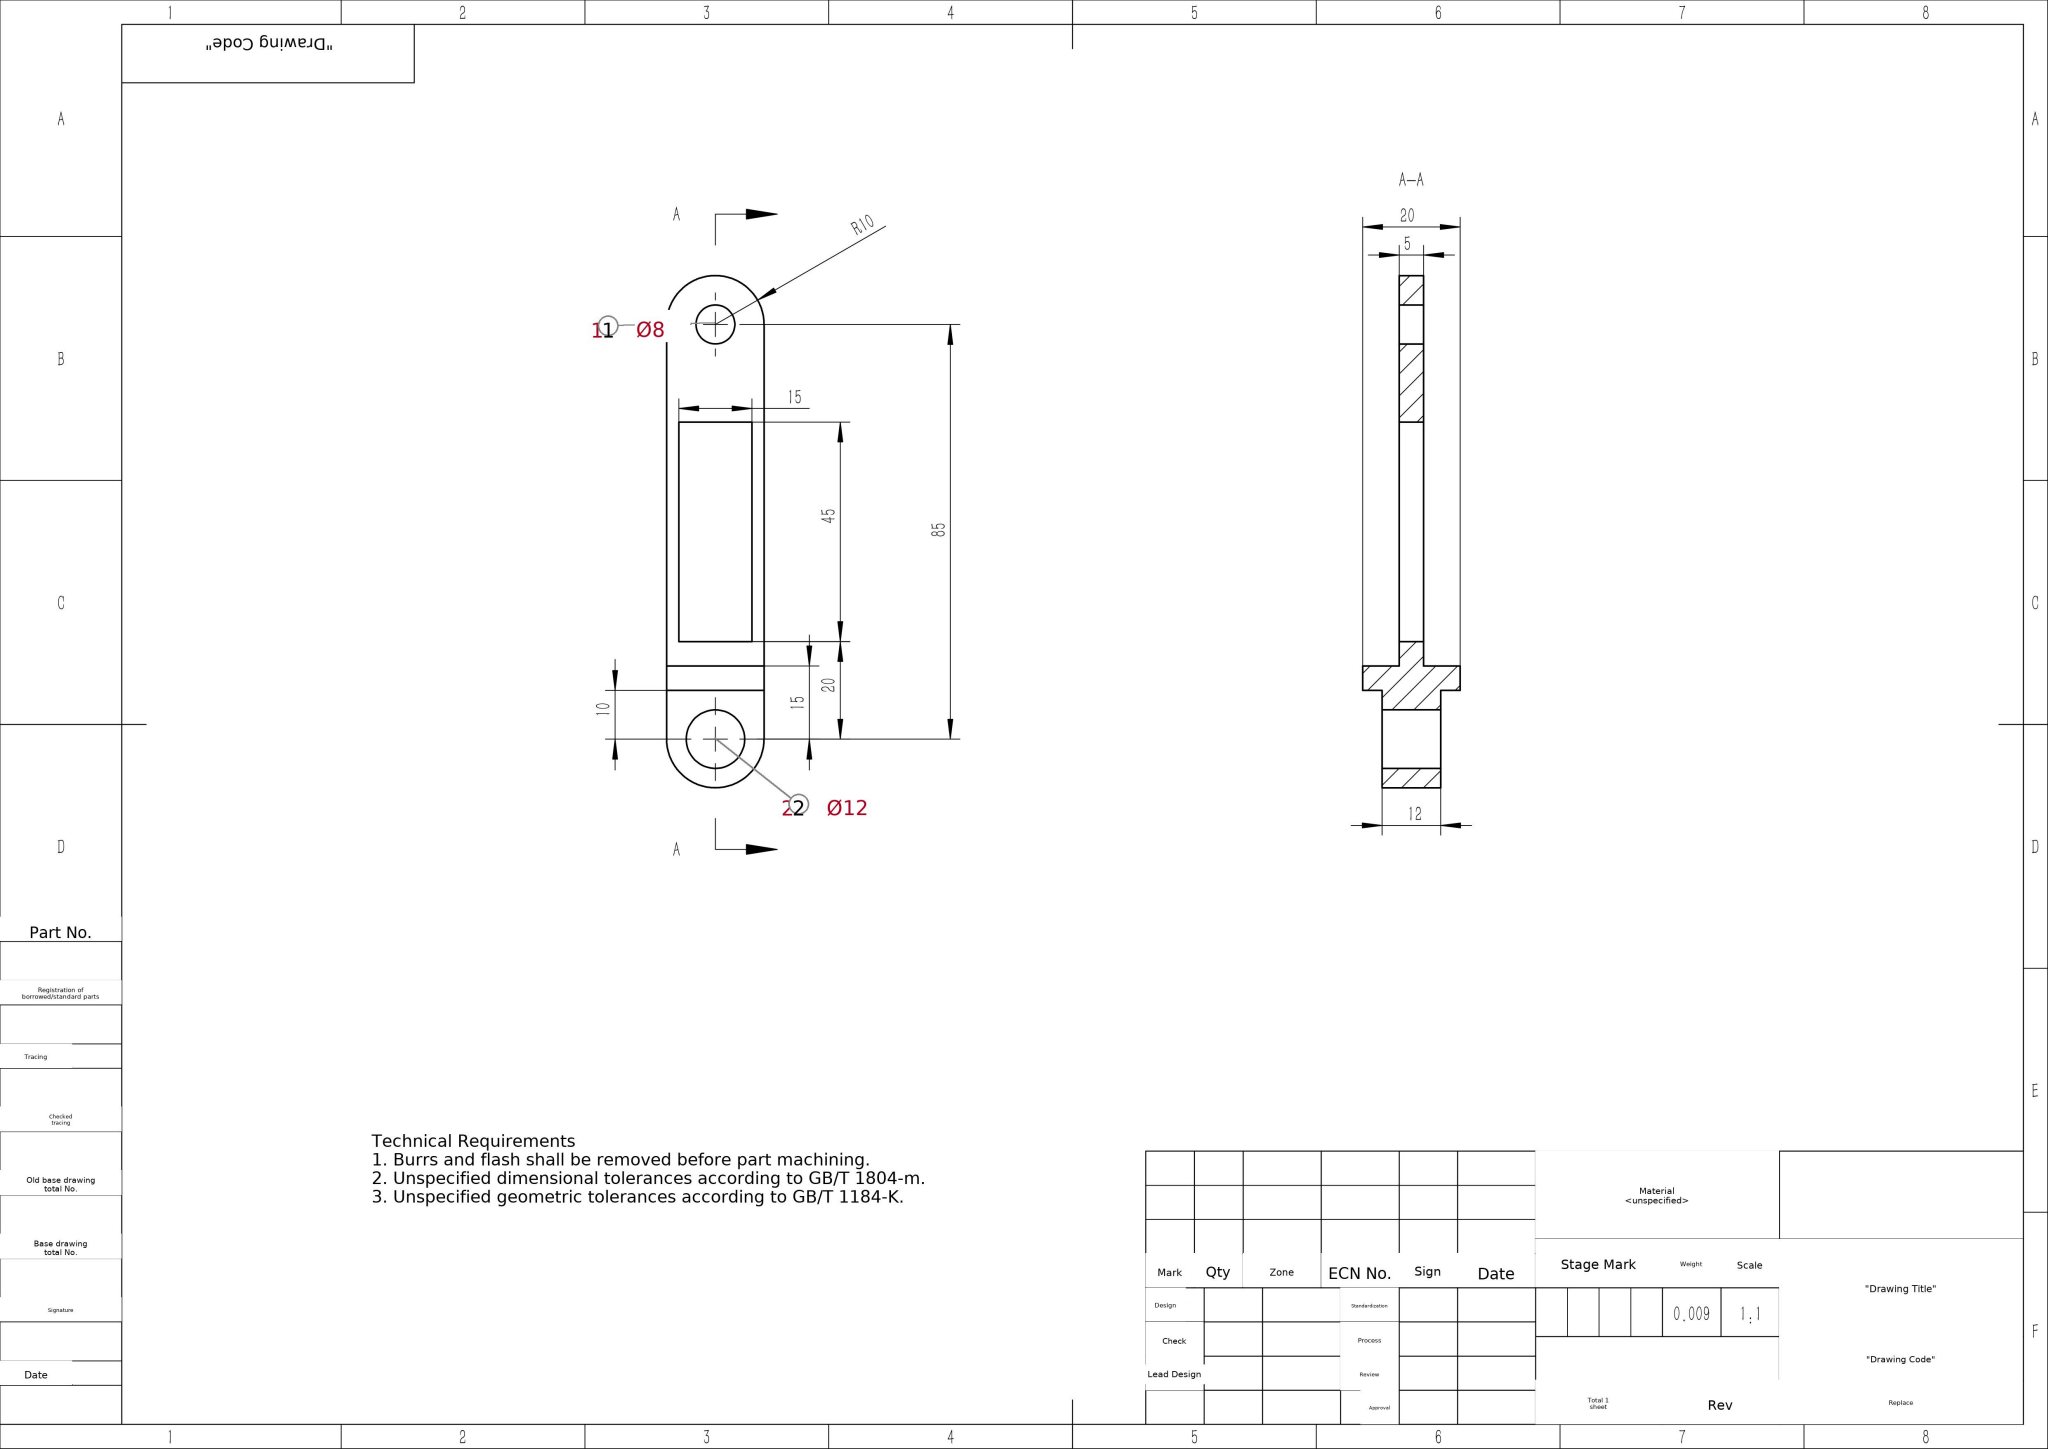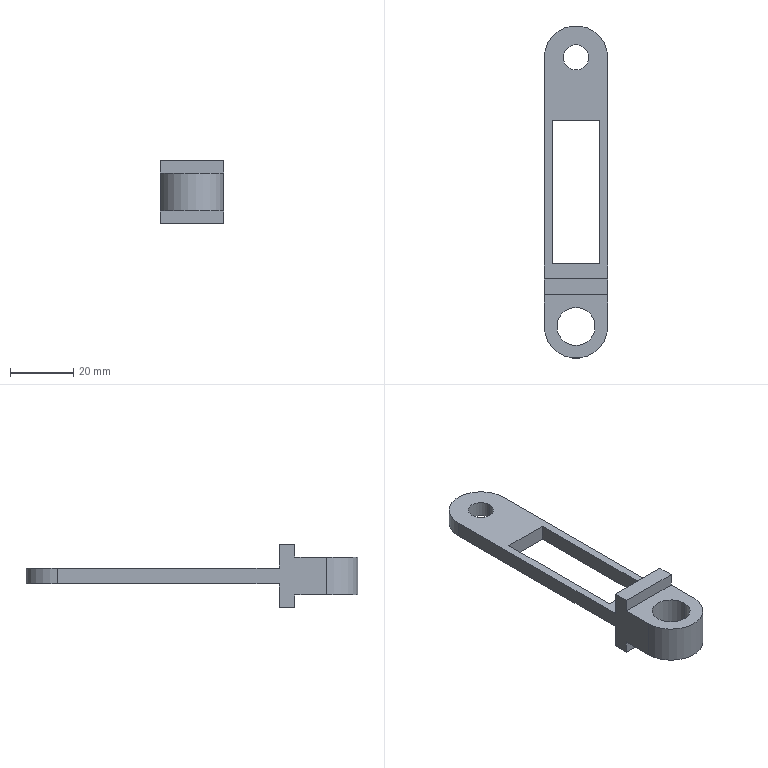Part | SolidWorks | mm | 1 solid | 22 faces | box 20 x 105 x 20 mm | volume 9087 mm3 | plane 16 | cylinder 6 | commonest cylinder face diameters 12 x2 8 x2 20 x2
build123d program:
from build123d import *

# Parameters (mm, degrees)
SKETCH1_W           = 20
SKETCH1_H           = 20
BOSS_EXTRUDE1_DEPTH = 5
SKETCH2_R           = 4
SKETCH2_W           = 15
SKETCH2_H           = 45
BOSS_EXTRUDE2_DEPTH = 2.5
SKETCH3_R           = 6
BOSS_EXTRUDE3_DEPTH = 6


with BuildPart() as part:
    # Sketch1 → Boss-Extrude1 (new body)
    with BuildSketch(Plane(origin=(0, 0, 0), x_dir=(1, 0, 0), z_dir=(0, 1, 0))):
        Rectangle(SKETCH1_W, SKETCH1_H)
    extrude(amount=BOSS_EXTRUDE1_DEPTH)

    # Sketch2 → Boss-Extrude2 (add, symmetric)
    with BuildSketch(Plane.XY):
        with BuildLine():
            Line((-10, 5), (10, 5))
            Line((10, 5), (10, 75))
            ThreePointArc((10, 75), (0, 85), (-10, 75))
            Line((-10, 75), (-10, 5))
        make_face()
        with Locations((0, 75)):
            Circle(SKETCH2_R, mode=Mode.SUBTRACT)
        with Locations((0, 32.5)):
            Rectangle(SKETCH2_W, SKETCH2_H, mode=Mode.SUBTRACT)
    extrude(amount=BOSS_EXTRUDE2_DEPTH, both=True)

    # Sketch3 → Boss-Extrude3 (add, symmetric)
    with BuildSketch(Plane.XY):
        with BuildLine():
            Line((-10, 0), (10, 0))
            Line((10, 0), (10, -10))
            ThreePointArc((10, -10), (0, -20), (-10, -10))
            Line((-10, -10), (-10, 0))
        make_face()
        with Locations((0, -10)):
            Circle(SKETCH3_R, mode=Mode.SUBTRACT)
    extrude(amount=BOSS_EXTRUDE3_DEPTH, both=True)


solid = part.part
STEP:
#1=CARTESIAN_POINT('',(-6.,-10.,6.));
#2=VERTEX_POINT('',#1);
#3=CARTESIAN_POINT('',(6.,-10.,6.));
#4=VERTEX_POINT('',#3);
#5=CARTESIAN_POINT('',(0.,-10.,6.));
#6=DIRECTION('',(0.,0.,1.));
#7=DIRECTION('',(1.,0.,0.));
#8=AXIS2_PLACEMENT_3D('',#5,#6,#7);
#9=CIRCLE('',#8,6.);
#10=EDGE_CURVE('',#2,#4,#9,.T.);
#11=ORIENTED_EDGE('',*,*,#10,.T.);
#12=CARTESIAN_POINT('',(6.,-10.,-6.));
#13=VERTEX_POINT('',#12);
#14=CARTESIAN_POINT('',(6.,-10.,6.));
#15=DIRECTION('',(0.,0.,-1.));
#16=VECTOR('',#15,1000.);
#17=LINE('',#14,#16);
#18=EDGE_CURVE('',#4,#13,#17,.T.);
#19=ORIENTED_EDGE('',*,*,#18,.T.);
#20=CARTESIAN_POINT('',(-6.,-10.,-6.));
#21=VERTEX_POINT('',#20);
#22=CARTESIAN_POINT('',(0.,-10.,-6.));
#23=DIRECTION('',(0.,0.,1.));
#24=DIRECTION('',(1.,0.,0.));
#25=AXIS2_PLACEMENT_3D('',#22,#23,#24);
#26=CIRCLE('',#25,6.);
#27=EDGE_CURVE('',#21,#13,#26,.T.);
#28=ORIENTED_EDGE('',*,*,#27,.F.);
#29=CARTESIAN_POINT('',(-6.,-10.,6.));
#30=DIRECTION('',(0.,0.,-1.));
#31=VECTOR('',#30,1000.);
#32=LINE('',#29,#31);
#33=EDGE_CURVE('',#2,#21,#32,.T.);
#34=ORIENTED_EDGE('',*,*,#33,.F.);
#35=EDGE_LOOP('',(#11,#19,#28,#34));
#36=FACE_OUTER_BOUND('',#35,.T.);
#37=CARTESIAN_POINT('',(0.,-10.,6.));
#38=DIRECTION('',(0.,0.,-1.));
#39=DIRECTION('',(-1.,0.,0.));
#40=AXIS2_PLACEMENT_3D('',#37,#38,#39);
#41=CYLINDRICAL_SURFACE('',#40,6.);
#42=ADVANCED_FACE('',(#36),#41,.F.);
#43=CARTESIAN_POINT('',(-4.,75.,2.5));
#44=VERTEX_POINT('',#43);
#45=CARTESIAN_POINT('',(4.,75.,2.5));
#46=VERTEX_POINT('',#45);
#47=CARTESIAN_POINT('',(0.,75.,2.5));
#48=DIRECTION('',(0.,0.,1.));
#49=DIRECTION('',(1.,0.,0.));
#50=AXIS2_PLACEMENT_3D('',#47,#48,#49);
#51=CIRCLE('',#50,4.);
#52=EDGE_CURVE('',#44,#46,#51,.T.);
#53=ORIENTED_EDGE('',*,*,#52,.T.);
#54=CARTESIAN_POINT('',(4.,75.,-2.5));
#55=VERTEX_POINT('',#54);
#56=CARTESIAN_POINT('',(4.,75.,2.5));
#57=DIRECTION('',(0.,0.,-1.));
#58=VECTOR('',#57,1000.);
#59=LINE('',#56,#58);
#60=EDGE_CURVE('',#46,#55,#59,.T.);
#61=ORIENTED_EDGE('',*,*,#60,.T.);
#62=CARTESIAN_POINT('',(-4.,75.,-2.5));
#63=VERTEX_POINT('',#62);
#64=CARTESIAN_POINT('',(0.,75.,-2.5));
#65=DIRECTION('',(0.,0.,1.));
#66=DIRECTION('',(1.,0.,0.));
#67=AXIS2_PLACEMENT_3D('',#64,#65,#66);
#68=CIRCLE('',#67,4.);
#69=EDGE_CURVE('',#63,#55,#68,.T.);
#70=ORIENTED_EDGE('',*,*,#69,.F.);
#71=CARTESIAN_POINT('',(-4.,75.,2.5));
#72=DIRECTION('',(0.,0.,-1.));
#73=VECTOR('',#72,1000.);
#74=LINE('',#71,#73);
#75=EDGE_CURVE('',#44,#63,#74,.T.);
#76=ORIENTED_EDGE('',*,*,#75,.F.);
#77=EDGE_LOOP('',(#53,#61,#70,#76));
#78=FACE_OUTER_BOUND('',#77,.T.);
#79=CARTESIAN_POINT('',(0.,75.,2.5));
#80=DIRECTION('',(0.,0.,-1.));
#81=DIRECTION('',(-1.,0.,0.));
#82=AXIS2_PLACEMENT_3D('',#79,#80,#81);
#83=CYLINDRICAL_SURFACE('',#82,4.);
#84=ADVANCED_FACE('',(#78),#83,.F.);
#85=CARTESIAN_POINT('',(10.,0.,6.));
#86=VERTEX_POINT('',#85);
#87=CARTESIAN_POINT('',(-10.,0.,6.));
#88=VERTEX_POINT('',#87);
#89=CARTESIAN_POINT('',(-10.,0.,6.));
#90=DIRECTION('',(-1.,0.,0.));
#91=VECTOR('',#90,1000.);
#92=LINE('',#89,#91);
#93=EDGE_CURVE('',#86,#88,#92,.T.);
#94=ORIENTED_EDGE('',*,*,#93,.F.);
#95=CARTESIAN_POINT('',(10.,0.,10.));
#96=VERTEX_POINT('',#95);
#97=CARTESIAN_POINT('',(10.,0.,-10.));
#98=DIRECTION('',(-0.,0.,-1.));
#99=VECTOR('',#98,1000.);
#100=LINE('',#97,#99);
#101=EDGE_CURVE('',#96,#86,#100,.T.);
#102=ORIENTED_EDGE('',*,*,#101,.F.);
#103=CARTESIAN_POINT('',(-10.,0.,10.));
#104=VERTEX_POINT('',#103);
#105=CARTESIAN_POINT('',(-10.,0.,10.));
#106=DIRECTION('',(1.,0.,0.));
#107=VECTOR('',#106,1000.);
#108=LINE('',#105,#107);
#109=EDGE_CURVE('',#104,#96,#108,.T.);
#110=ORIENTED_EDGE('',*,*,#109,.F.);
#111=CARTESIAN_POINT('',(-10.,0.,-10.));
#112=DIRECTION('',(0.,0.,1.));
#113=VECTOR('',#112,1000.);
#114=LINE('',#111,#113);
#115=EDGE_CURVE('',#88,#104,#114,.T.);
#116=ORIENTED_EDGE('',*,*,#115,.F.);
#117=EDGE_LOOP('',(#94,#102,#110,#116));
#118=FACE_OUTER_BOUND('',#117,.T.);
#119=CARTESIAN_POINT('',(0.,0.,0.));
#120=DIRECTION('',(0.,1.,0.));
#121=DIRECTION('',(0.,0.,1.));
#122=AXIS2_PLACEMENT_3D('',#119,#120,#121);
#123=PLANE('',#122);
#124=ADVANCED_FACE('',(#118),#123,.F.);
#125=CARTESIAN_POINT('',(-10.,5.,-10.));
#126=VERTEX_POINT('',#125);
#127=CARTESIAN_POINT('',(-10.,5.,-2.5));
#128=VERTEX_POINT('',#127);
#129=CARTESIAN_POINT('',(-10.,5.,-10.));
#130=DIRECTION('',(0.,0.,1.));
#131=VECTOR('',#130,1000.);
#132=LINE('',#129,#131);
#133=EDGE_CURVE('',#126,#128,#132,.T.);
#134=ORIENTED_EDGE('',*,*,#133,.T.);
#135=CARTESIAN_POINT('',(10.,5.,-2.5));
#136=VERTEX_POINT('',#135);
#137=CARTESIAN_POINT('',(-10.,5.,-2.5));
#138=DIRECTION('',(1.,0.,0.));
#139=VECTOR('',#138,1000.);
#140=LINE('',#137,#139);
#141=EDGE_CURVE('',#128,#136,#140,.T.);
#142=ORIENTED_EDGE('',*,*,#141,.T.);
#143=CARTESIAN_POINT('',(10.,5.,-10.));
#144=VERTEX_POINT('',#143);
#145=CARTESIAN_POINT('',(10.,5.,-10.));
#146=DIRECTION('',(-0.,0.,-1.));
#147=VECTOR('',#146,1000.);
#148=LINE('',#145,#147);
#149=EDGE_CURVE('',#136,#144,#148,.T.);
#150=ORIENTED_EDGE('',*,*,#149,.T.);
#151=CARTESIAN_POINT('',(-10.,5.,-10.));
#152=DIRECTION('',(-1.,0.,0.));
#153=VECTOR('',#152,1000.);
#154=LINE('',#151,#153);
#155=EDGE_CURVE('',#144,#126,#154,.T.);
#156=ORIENTED_EDGE('',*,*,#155,.T.);
#157=EDGE_LOOP('',(#134,#142,#150,#156));
#158=FACE_OUTER_BOUND('',#157,.T.);
#159=CARTESIAN_POINT('',(0.,5.,0.));
#160=DIRECTION('',(0.,1.,0.));
#161=DIRECTION('',(0.,0.,1.));
#162=AXIS2_PLACEMENT_3D('',#159,#160,#161);
#163=PLANE('',#162);
#164=ADVANCED_FACE('',(#158),#163,.T.);
#165=ORIENTED_EDGE('',*,*,#101,.T.);
#166=CARTESIAN_POINT('',(10.,-10.,6.));
#167=VERTEX_POINT('',#166);
#168=CARTESIAN_POINT('',(10.,0.,6.));
#169=DIRECTION('',(-0.,1.,0.));
#170=VECTOR('',#169,1000.);
#171=LINE('',#168,#170);
#172=EDGE_CURVE('',#167,#86,#171,.T.);
#173=ORIENTED_EDGE('',*,*,#172,.F.);
#174=CARTESIAN_POINT('',(10.,-10.,-6.));
#175=VERTEX_POINT('',#174);
#176=CARTESIAN_POINT('',(10.,-10.,6.));
#177=DIRECTION('',(0.,0.,-1.));
#178=VECTOR('',#177,1000.);
#179=LINE('',#176,#178);
#180=EDGE_CURVE('',#167,#175,#179,.T.);
#181=ORIENTED_EDGE('',*,*,#180,.T.);
#182=CARTESIAN_POINT('',(10.,0.,-6.));
#183=VERTEX_POINT('',#182);
#184=CARTESIAN_POINT('',(10.,0.,-6.));
#185=DIRECTION('',(-0.,1.,0.));
#186=VECTOR('',#185,1000.);
#187=LINE('',#184,#186);
#188=EDGE_CURVE('',#175,#183,#187,.T.);
#189=ORIENTED_EDGE('',*,*,#188,.T.);
#190=CARTESIAN_POINT('',(10.,0.,-10.));
#191=VERTEX_POINT('',#190);
#192=CARTESIAN_POINT('',(10.,0.,-10.));
#193=DIRECTION('',(-0.,0.,-1.));
#194=VECTOR('',#193,1000.);
#195=LINE('',#192,#194);
#196=EDGE_CURVE('',#183,#191,#195,.T.);
#197=ORIENTED_EDGE('',*,*,#196,.T.);
#198=CARTESIAN_POINT('',(10.,5.,-10.));
#199=DIRECTION('',(0.,-1.,0.));
#200=VECTOR('',#199,1000.);
#201=LINE('',#198,#200);
#202=EDGE_CURVE('',#144,#191,#201,.T.);
#203=ORIENTED_EDGE('',*,*,#202,.F.);
#204=ORIENTED_EDGE('',*,*,#149,.F.);
#205=CARTESIAN_POINT('',(10.,75.,-2.5));
#206=VERTEX_POINT('',#205);
#207=CARTESIAN_POINT('',(10.,5.,-2.5));
#208=DIRECTION('',(0.,1.,0.));
#209=VECTOR('',#208,1000.);
#210=LINE('',#207,#209);
#211=EDGE_CURVE('',#136,#206,#210,.T.);
#212=ORIENTED_EDGE('',*,*,#211,.T.);
#213=CARTESIAN_POINT('',(10.,75.,2.5));
#214=VERTEX_POINT('',#213);
#215=CARTESIAN_POINT('',(10.,75.,2.5));
#216=DIRECTION('',(0.,0.,-1.));
#217=VECTOR('',#216,1000.);
#218=LINE('',#215,#217);
#219=EDGE_CURVE('',#214,#206,#218,.T.);
#220=ORIENTED_EDGE('',*,*,#219,.F.);
#221=CARTESIAN_POINT('',(10.,5.,2.5));
#222=VERTEX_POINT('',#221);
#223=CARTESIAN_POINT('',(10.,5.,2.5));
#224=DIRECTION('',(0.,1.,0.));
#225=VECTOR('',#224,1000.);
#226=LINE('',#223,#225);
#227=EDGE_CURVE('',#222,#214,#226,.T.);
#228=ORIENTED_EDGE('',*,*,#227,.F.);
#229=CARTESIAN_POINT('',(10.,5.,10.));
#230=VERTEX_POINT('',#229);
#231=CARTESIAN_POINT('',(10.,5.,-10.));
#232=DIRECTION('',(-0.,0.,-1.));
#233=VECTOR('',#232,1000.);
#234=LINE('',#231,#233);
#235=EDGE_CURVE('',#230,#222,#234,.T.);
#236=ORIENTED_EDGE('',*,*,#235,.F.);
#237=CARTESIAN_POINT('',(10.,5.,10.));
#238=DIRECTION('',(0.,-1.,0.));
#239=VECTOR('',#238,1000.);
#240=LINE('',#237,#239);
#241=EDGE_CURVE('',#230,#96,#240,.T.);
#242=ORIENTED_EDGE('',*,*,#241,.T.);
#243=EDGE_LOOP('',(#165,#173,#181,#189,#197,#203,#204,#212,#220,#228,#236,#242));
#244=FACE_OUTER_BOUND('',#243,.T.);
#245=CARTESIAN_POINT('',(10.,5.,-10.));
#246=DIRECTION('',(-1.,0.,0.));
#247=DIRECTION('',(0.,0.,1.));
#248=AXIS2_PLACEMENT_3D('',#245,#246,#247);
#249=PLANE('',#248);
#250=ADVANCED_FACE('',(#244),#249,.F.);
#251=CARTESIAN_POINT('',(-10.,0.,-10.));
#252=VERTEX_POINT('',#251);
#253=CARTESIAN_POINT('',(-10.,0.,-10.));
#254=DIRECTION('',(-1.,0.,0.));
#255=VECTOR('',#254,1000.);
#256=LINE('',#253,#255);
#257=EDGE_CURVE('',#191,#252,#256,.T.);
#258=ORIENTED_EDGE('',*,*,#257,.T.);
#259=CARTESIAN_POINT('',(-10.,5.,-10.));
#260=DIRECTION('',(0.,-1.,0.));
#261=VECTOR('',#260,1000.);
#262=LINE('',#259,#261);
#263=EDGE_CURVE('',#126,#252,#262,.T.);
#264=ORIENTED_EDGE('',*,*,#263,.F.);
#265=ORIENTED_EDGE('',*,*,#155,.F.);
#266=ORIENTED_EDGE('',*,*,#202,.T.);
#267=EDGE_LOOP('',(#258,#264,#265,#266));
#268=FACE_OUTER_BOUND('',#267,.T.);
#269=CARTESIAN_POINT('',(-10.,5.,-10.));
#270=DIRECTION('',(0.,0.,1.));
#271=DIRECTION('',(1.,0.,0.));
#272=AXIS2_PLACEMENT_3D('',#269,#270,#271);
#273=PLANE('',#272);
#274=ADVANCED_FACE('',(#268),#273,.F.);
#275=CARTESIAN_POINT('',(-10.,0.,-6.));
#276=VERTEX_POINT('',#275);
#277=CARTESIAN_POINT('',(-10.,0.,-10.));
#278=DIRECTION('',(0.,0.,1.));
#279=VECTOR('',#278,1000.);
#280=LINE('',#277,#279);
#281=EDGE_CURVE('',#252,#276,#280,.T.);
#282=ORIENTED_EDGE('',*,*,#281,.T.);
#283=CARTESIAN_POINT('',(-10.,-10.,-6.));
#284=VERTEX_POINT('',#283);
#285=CARTESIAN_POINT('',(-10.,0.,-6.));
#286=DIRECTION('',(0.,-1.,0.));
#287=VECTOR('',#286,1000.);
#288=LINE('',#285,#287);
#289=EDGE_CURVE('',#276,#284,#288,.T.);
#290=ORIENTED_EDGE('',*,*,#289,.T.);
#291=CARTESIAN_POINT('',(-10.,-10.,6.));
#292=VERTEX_POINT('',#291);
#293=CARTESIAN_POINT('',(-10.,-10.,6.));
#294=DIRECTION('',(0.,0.,-1.));
#295=VECTOR('',#294,1000.);
#296=LINE('',#293,#295);
#297=EDGE_CURVE('',#292,#284,#296,.T.);
#298=ORIENTED_EDGE('',*,*,#297,.F.);
#299=CARTESIAN_POINT('',(-10.,0.,6.));
#300=DIRECTION('',(0.,-1.,0.));
#301=VECTOR('',#300,1000.);
#302=LINE('',#299,#301);
#303=EDGE_CURVE('',#88,#292,#302,.T.);
#304=ORIENTED_EDGE('',*,*,#303,.F.);
#305=ORIENTED_EDGE('',*,*,#115,.T.);
#306=CARTESIAN_POINT('',(-10.,5.,10.));
#307=VERTEX_POINT('',#306);
#308=CARTESIAN_POINT('',(-10.,5.,10.));
#309=DIRECTION('',(0.,-1.,0.));
#310=VECTOR('',#309,1000.);
#311=LINE('',#308,#310);
#312=EDGE_CURVE('',#307,#104,#311,.T.);
#313=ORIENTED_EDGE('',*,*,#312,.F.);
#314=CARTESIAN_POINT('',(-10.,5.,2.5));
#315=VERTEX_POINT('',#314);
#316=CARTESIAN_POINT('',(-10.,5.,-10.));
#317=DIRECTION('',(0.,0.,1.));
#318=VECTOR('',#317,1000.);
#319=LINE('',#316,#318);
#320=EDGE_CURVE('',#315,#307,#319,.T.);
#321=ORIENTED_EDGE('',*,*,#320,.F.);
#322=CARTESIAN_POINT('',(-10.,75.,2.5));
#323=VERTEX_POINT('',#322);
#324=CARTESIAN_POINT('',(-10.,5.,2.5));
#325=DIRECTION('',(0.,-1.,0.));
#326=VECTOR('',#325,1000.);
#327=LINE('',#324,#326);
#328=EDGE_CURVE('',#323,#315,#327,.T.);
#329=ORIENTED_EDGE('',*,*,#328,.F.);
#330=CARTESIAN_POINT('',(-10.,75.,-2.5));
#331=VERTEX_POINT('',#330);
#332=CARTESIAN_POINT('',(-10.,75.,2.5));
#333=DIRECTION('',(0.,0.,-1.));
#334=VECTOR('',#333,1000.);
#335=LINE('',#332,#334);
#336=EDGE_CURVE('',#323,#331,#335,.T.);
#337=ORIENTED_EDGE('',*,*,#336,.T.);
#338=CARTESIAN_POINT('',(-10.,5.,-2.5));
#339=DIRECTION('',(0.,-1.,0.));
#340=VECTOR('',#339,1000.);
#341=LINE('',#338,#340);
#342=EDGE_CURVE('',#331,#128,#341,.T.);
#343=ORIENTED_EDGE('',*,*,#342,.T.);
#344=ORIENTED_EDGE('',*,*,#133,.F.);
#345=ORIENTED_EDGE('',*,*,#263,.T.);
#346=EDGE_LOOP('',(#282,#290,#298,#304,#305,#313,#321,#329,#337,#343,#344,#345));
#347=FACE_OUTER_BOUND('',#346,.T.);
#348=CARTESIAN_POINT('',(-10.,5.,-10.));
#349=DIRECTION('',(1.,0.,-0.));
#350=DIRECTION('',(-0.,0.,-1.));
#351=AXIS2_PLACEMENT_3D('',#348,#349,#350);
#352=PLANE('',#351);
#353=ADVANCED_FACE('',(#347),#352,.F.);
#354=ORIENTED_EDGE('',*,*,#109,.T.);
#355=ORIENTED_EDGE('',*,*,#241,.F.);
#356=CARTESIAN_POINT('',(-10.,5.,10.));
#357=DIRECTION('',(1.,0.,0.));
#358=VECTOR('',#357,1000.);
#359=LINE('',#356,#358);
#360=EDGE_CURVE('',#307,#230,#359,.T.);
#361=ORIENTED_EDGE('',*,*,#360,.F.);
#362=ORIENTED_EDGE('',*,*,#312,.T.);
#363=EDGE_LOOP('',(#354,#355,#361,#362));
#364=FACE_OUTER_BOUND('',#363,.T.);
#365=CARTESIAN_POINT('',(-10.,5.,10.));
#366=DIRECTION('',(0.,0.,-1.));
#367=DIRECTION('',(-1.,0.,0.));
#368=AXIS2_PLACEMENT_3D('',#365,#366,#367);
#369=PLANE('',#368);
#370=ADVANCED_FACE('',(#364),#369,.F.);
#371=CARTESIAN_POINT('',(-10.,5.,2.5));
#372=DIRECTION('',(1.,0.,0.));
#373=VECTOR('',#372,1000.);
#374=LINE('',#371,#373);
#375=EDGE_CURVE('',#315,#222,#374,.T.);
#376=ORIENTED_EDGE('',*,*,#375,.F.);
#377=ORIENTED_EDGE('',*,*,#320,.T.);
#378=ORIENTED_EDGE('',*,*,#360,.T.);
#379=ORIENTED_EDGE('',*,*,#235,.T.);
#380=EDGE_LOOP('',(#376,#377,#378,#379));
#381=FACE_OUTER_BOUND('',#380,.T.);
#382=CARTESIAN_POINT('',(0.,5.,0.));
#383=DIRECTION('',(0.,1.,0.));
#384=DIRECTION('',(0.,0.,1.));
#385=AXIS2_PLACEMENT_3D('',#382,#383,#384);
#386=PLANE('',#385);
#387=ADVANCED_FACE('',(#381),#386,.T.);
#388=ORIENTED_EDGE('',*,*,#196,.F.);
#389=CARTESIAN_POINT('',(-10.,0.,-6.));
#390=DIRECTION('',(-1.,0.,0.));
#391=VECTOR('',#390,1000.);
#392=LINE('',#389,#391);
#393=EDGE_CURVE('',#183,#276,#392,.T.);
#394=ORIENTED_EDGE('',*,*,#393,.T.);
#395=ORIENTED_EDGE('',*,*,#281,.F.);
#396=ORIENTED_EDGE('',*,*,#257,.F.);
#397=EDGE_LOOP('',(#388,#394,#395,#396));
#398=FACE_OUTER_BOUND('',#397,.T.);
#399=CARTESIAN_POINT('',(0.,0.,0.));
#400=DIRECTION('',(0.,1.,0.));
#401=DIRECTION('',(0.,0.,1.));
#402=AXIS2_PLACEMENT_3D('',#399,#400,#401);
#403=PLANE('',#402);
#404=ADVANCED_FACE('',(#398),#403,.F.);
#405=CARTESIAN_POINT('',(-7.5,10.,2.5));
#406=VERTEX_POINT('',#405);
#407=CARTESIAN_POINT('',(7.5,10.,2.5));
#408=VERTEX_POINT('',#407);
#409=CARTESIAN_POINT('',(-7.5,10.,2.5));
#410=DIRECTION('',(1.,0.,0.));
#411=VECTOR('',#410,1000.);
#412=LINE('',#409,#411);
#413=EDGE_CURVE('',#406,#408,#412,.T.);
#414=ORIENTED_EDGE('',*,*,#413,.F.);
#415=CARTESIAN_POINT('',(-7.5,55.,2.5));
#416=VERTEX_POINT('',#415);
#417=CARTESIAN_POINT('',(-7.5,10.,2.5));
#418=DIRECTION('',(0.,-1.,0.));
#419=VECTOR('',#418,1000.);
#420=LINE('',#417,#419);
#421=EDGE_CURVE('',#416,#406,#420,.T.);
#422=ORIENTED_EDGE('',*,*,#421,.F.);
#423=CARTESIAN_POINT('',(7.5,55.,2.5));
#424=VERTEX_POINT('',#423);
#425=CARTESIAN_POINT('',(-7.5,55.,2.5));
#426=DIRECTION('',(-1.,0.,0.));
#427=VECTOR('',#426,1000.);
#428=LINE('',#425,#427);
#429=EDGE_CURVE('',#424,#416,#428,.T.);
#430=ORIENTED_EDGE('',*,*,#429,.F.);
#431=CARTESIAN_POINT('',(7.5,10.,2.5));
#432=DIRECTION('',(0.,1.,0.));
#433=VECTOR('',#432,1000.);
#434=LINE('',#431,#433);
#435=EDGE_CURVE('',#408,#424,#434,.T.);
#436=ORIENTED_EDGE('',*,*,#435,.F.);
#437=EDGE_LOOP('',(#414,#422,#430,#436));
#438=FACE_BOUND('',#437,.T.);
#439=ORIENTED_EDGE('',*,*,#328,.T.);
#440=ORIENTED_EDGE('',*,*,#375,.T.);
#441=ORIENTED_EDGE('',*,*,#227,.T.);
#442=CARTESIAN_POINT('',(0.,75.,2.5));
#443=DIRECTION('',(0.,0.,1.));
#444=DIRECTION('',(1.,0.,0.));
#445=AXIS2_PLACEMENT_3D('',#442,#443,#444);
#446=CIRCLE('',#445,10.);
#447=EDGE_CURVE('',#214,#323,#446,.T.);
#448=ORIENTED_EDGE('',*,*,#447,.T.);
#449=EDGE_LOOP('',(#439,#440,#441,#448));
#450=FACE_OUTER_BOUND('',#449,.T.);
#451=ORIENTED_EDGE('',*,*,#52,.F.);
#452=CARTESIAN_POINT('',(0.,75.,2.5));
#453=DIRECTION('',(0.,0.,1.));
#454=DIRECTION('',(1.,0.,0.));
#455=AXIS2_PLACEMENT_3D('',#452,#453,#454);
#456=CIRCLE('',#455,4.);
#457=EDGE_CURVE('',#46,#44,#456,.T.);
#458=ORIENTED_EDGE('',*,*,#457,.F.);
#459=EDGE_LOOP('',(#451,#458));
#460=FACE_BOUND('',#459,.T.);
#461=CARTESIAN_POINT('',(0.,75.,2.5));
#462=DIRECTION('',(0.,0.,1.));
#463=DIRECTION('',(1.,0.,0.));
#464=AXIS2_PLACEMENT_3D('',#461,#462,#463);
#465=PLANE('',#464);
#466=ADVANCED_FACE('',(#438,#450,#460),#465,.T.);
#467=ORIENTED_EDGE('',*,*,#342,.F.);
#468=CARTESIAN_POINT('',(0.,75.,-2.5));
#469=DIRECTION('',(0.,0.,1.));
#470=DIRECTION('',(1.,0.,0.));
#471=AXIS2_PLACEMENT_3D('',#468,#469,#470);
#472=CIRCLE('',#471,10.);
#473=EDGE_CURVE('',#206,#331,#472,.T.);
#474=ORIENTED_EDGE('',*,*,#473,.F.);
#475=ORIENTED_EDGE('',*,*,#211,.F.);
#476=ORIENTED_EDGE('',*,*,#141,.F.);
#477=EDGE_LOOP('',(#467,#474,#475,#476));
#478=FACE_OUTER_BOUND('',#477,.T.);
#479=CARTESIAN_POINT('',(-7.5,55.,-2.5));
#480=VERTEX_POINT('',#479);
#481=CARTESIAN_POINT('',(-7.5,10.,-2.5));
#482=VERTEX_POINT('',#481);
#483=CARTESIAN_POINT('',(-7.5,10.,-2.5));
#484=DIRECTION('',(0.,-1.,0.));
#485=VECTOR('',#484,1000.);
#486=LINE('',#483,#485);
#487=EDGE_CURVE('',#480,#482,#486,.T.);
#488=ORIENTED_EDGE('',*,*,#487,.T.);
#489=CARTESIAN_POINT('',(7.5,10.,-2.5));
#490=VERTEX_POINT('',#489);
#491=CARTESIAN_POINT('',(-7.5,10.,-2.5));
#492=DIRECTION('',(1.,0.,0.));
#493=VECTOR('',#492,1000.);
#494=LINE('',#491,#493);
#495=EDGE_CURVE('',#482,#490,#494,.T.);
#496=ORIENTED_EDGE('',*,*,#495,.T.);
#497=CARTESIAN_POINT('',(7.5,55.,-2.5));
#498=VERTEX_POINT('',#497);
#499=CARTESIAN_POINT('',(7.5,10.,-2.5));
#500=DIRECTION('',(0.,1.,0.));
#501=VECTOR('',#500,1000.);
#502=LINE('',#499,#501);
#503=EDGE_CURVE('',#490,#498,#502,.T.);
#504=ORIENTED_EDGE('',*,*,#503,.T.);
#505=CARTESIAN_POINT('',(-7.5,55.,-2.5));
#506=DIRECTION('',(-1.,0.,0.));
#507=VECTOR('',#506,1000.);
#508=LINE('',#505,#507);
#509=EDGE_CURVE('',#498,#480,#508,.T.);
#510=ORIENTED_EDGE('',*,*,#509,.T.);
#511=EDGE_LOOP('',(#488,#496,#504,#510));
#512=FACE_BOUND('',#511,.T.);
#513=ORIENTED_EDGE('',*,*,#69,.T.);
#514=CARTESIAN_POINT('',(0.,75.,-2.5));
#515=DIRECTION('',(0.,0.,1.));
#516=DIRECTION('',(1.,0.,0.));
#517=AXIS2_PLACEMENT_3D('',#514,#515,#516);
#518=CIRCLE('',#517,4.);
#519=EDGE_CURVE('',#55,#63,#518,.T.);
#520=ORIENTED_EDGE('',*,*,#519,.T.);
#521=EDGE_LOOP('',(#513,#520));
#522=FACE_BOUND('',#521,.T.);
#523=CARTESIAN_POINT('',(0.,75.,-2.5));
#524=DIRECTION('',(0.,0.,1.));
#525=DIRECTION('',(1.,0.,0.));
#526=AXIS2_PLACEMENT_3D('',#523,#524,#525);
#527=PLANE('',#526);
#528=ADVANCED_FACE('',(#478,#512,#522),#527,.F.);
#529=ORIENTED_EDGE('',*,*,#473,.T.);
#530=ORIENTED_EDGE('',*,*,#336,.F.);
#531=ORIENTED_EDGE('',*,*,#447,.F.);
#532=ORIENTED_EDGE('',*,*,#219,.T.);
#533=EDGE_LOOP('',(#529,#530,#531,#532));
#534=FACE_OUTER_BOUND('',#533,.T.);
#535=CARTESIAN_POINT('',(0.,75.,2.5));
#536=DIRECTION('',(0.,0.,-1.));
#537=DIRECTION('',(-1.,0.,0.));
#538=AXIS2_PLACEMENT_3D('',#535,#536,#537);
#539=CYLINDRICAL_SURFACE('',#538,10.);
#540=ADVANCED_FACE('',(#534),#539,.T.);
#541=ORIENTED_EDGE('',*,*,#487,.F.);
#542=CARTESIAN_POINT('',(-7.5,55.,2.5));
#543=DIRECTION('',(0.,0.,-1.));
#544=VECTOR('',#543,1000.);
#545=LINE('',#542,#544);
#546=EDGE_CURVE('',#416,#480,#545,.T.);
#547=ORIENTED_EDGE('',*,*,#546,.F.);
#548=ORIENTED_EDGE('',*,*,#421,.T.);
#549=CARTESIAN_POINT('',(-7.5,10.,2.5));
#550=DIRECTION('',(0.,0.,-1.));
#551=VECTOR('',#550,1000.);
#552=LINE('',#549,#551);
#553=EDGE_CURVE('',#406,#482,#552,.T.);
#554=ORIENTED_EDGE('',*,*,#553,.T.);
#555=EDGE_LOOP('',(#541,#547,#548,#554));
#556=FACE_OUTER_BOUND('',#555,.T.);
#557=CARTESIAN_POINT('',(-7.5,10.,2.5));
#558=DIRECTION('',(1.,0.,0.));
#559=DIRECTION('',(0.,0.,-1.));
#560=AXIS2_PLACEMENT_3D('',#557,#558,#559);
#561=PLANE('',#560);
#562=ADVANCED_FACE('',(#556),#561,.T.);
#563=ORIENTED_EDGE('',*,*,#495,.F.);
#564=ORIENTED_EDGE('',*,*,#553,.F.);
#565=ORIENTED_EDGE('',*,*,#413,.T.);
#566=CARTESIAN_POINT('',(7.5,10.,2.5));
#567=DIRECTION('',(0.,0.,-1.));
#568=VECTOR('',#567,1000.);
#569=LINE('',#566,#568);
#570=EDGE_CURVE('',#408,#490,#569,.T.);
#571=ORIENTED_EDGE('',*,*,#570,.T.);
#572=EDGE_LOOP('',(#563,#564,#565,#571));
#573=FACE_OUTER_BOUND('',#572,.T.);
#574=CARTESIAN_POINT('',(-7.5,10.,2.5));
#575=DIRECTION('',(0.,1.,0.));
#576=DIRECTION('',(0.,0.,1.));
#577=AXIS2_PLACEMENT_3D('',#574,#575,#576);
#578=PLANE('',#577);
#579=ADVANCED_FACE('',(#573),#578,.T.);
#580=ORIENTED_EDGE('',*,*,#503,.F.);
#581=ORIENTED_EDGE('',*,*,#570,.F.);
#582=ORIENTED_EDGE('',*,*,#435,.T.);
#583=CARTESIAN_POINT('',(7.5,55.,2.5));
#584=DIRECTION('',(0.,0.,-1.));
#585=VECTOR('',#584,1000.);
#586=LINE('',#583,#585);
#587=EDGE_CURVE('',#424,#498,#586,.T.);
#588=ORIENTED_EDGE('',*,*,#587,.T.);
#589=EDGE_LOOP('',(#580,#581,#582,#588));
#590=FACE_OUTER_BOUND('',#589,.T.);
#591=CARTESIAN_POINT('',(7.5,10.,2.5));
#592=DIRECTION('',(-1.,0.,0.));
#593=DIRECTION('',(0.,0.,1.));
#594=AXIS2_PLACEMENT_3D('',#591,#592,#593);
#595=PLANE('',#594);
#596=ADVANCED_FACE('',(#590),#595,.T.);
#597=ORIENTED_EDGE('',*,*,#509,.F.);
#598=ORIENTED_EDGE('',*,*,#587,.F.);
#599=ORIENTED_EDGE('',*,*,#429,.T.);
#600=ORIENTED_EDGE('',*,*,#546,.T.);
#601=EDGE_LOOP('',(#597,#598,#599,#600));
#602=FACE_OUTER_BOUND('',#601,.T.);
#603=CARTESIAN_POINT('',(-7.5,55.,2.5));
#604=DIRECTION('',(0.,-1.,0.));
#605=DIRECTION('',(0.,0.,-1.));
#606=AXIS2_PLACEMENT_3D('',#603,#604,#605);
#607=PLANE('',#606);
#608=ADVANCED_FACE('',(#602),#607,.T.);
#609=ORIENTED_EDGE('',*,*,#60,.F.);
#610=ORIENTED_EDGE('',*,*,#457,.T.);
#611=ORIENTED_EDGE('',*,*,#75,.T.);
#612=ORIENTED_EDGE('',*,*,#519,.F.);
#613=EDGE_LOOP('',(#609,#610,#611,#612));
#614=FACE_OUTER_BOUND('',#613,.T.);
#615=CARTESIAN_POINT('',(0.,75.,2.5));
#616=DIRECTION('',(0.,0.,-1.));
#617=DIRECTION('',(-1.,0.,0.));
#618=AXIS2_PLACEMENT_3D('',#615,#616,#617);
#619=CYLINDRICAL_SURFACE('',#618,4.);
#620=ADVANCED_FACE('',(#614),#619,.F.);
#621=ORIENTED_EDGE('',*,*,#303,.T.);
#622=CARTESIAN_POINT('',(0.,-10.,6.));
#623=DIRECTION('',(0.,0.,1.));
#624=DIRECTION('',(1.,0.,0.));
#625=AXIS2_PLACEMENT_3D('',#622,#623,#624);
#626=CIRCLE('',#625,10.);
#627=EDGE_CURVE('',#292,#167,#626,.T.);
#628=ORIENTED_EDGE('',*,*,#627,.T.);
#629=ORIENTED_EDGE('',*,*,#172,.T.);
#630=ORIENTED_EDGE('',*,*,#93,.T.);
#631=EDGE_LOOP('',(#621,#628,#629,#630));
#632=FACE_OUTER_BOUND('',#631,.T.);
#633=ORIENTED_EDGE('',*,*,#10,.F.);
#634=CARTESIAN_POINT('',(0.,-10.,6.));
#635=DIRECTION('',(0.,0.,1.));
#636=DIRECTION('',(1.,0.,0.));
#637=AXIS2_PLACEMENT_3D('',#634,#635,#636);
#638=CIRCLE('',#637,6.);
#639=EDGE_CURVE('',#4,#2,#638,.T.);
#640=ORIENTED_EDGE('',*,*,#639,.F.);
#641=EDGE_LOOP('',(#633,#640));
#642=FACE_BOUND('',#641,.T.);
#643=CARTESIAN_POINT('',(0.,-10.,6.));
#644=DIRECTION('',(0.,0.,1.));
#645=DIRECTION('',(1.,0.,0.));
#646=AXIS2_PLACEMENT_3D('',#643,#644,#645);
#647=PLANE('',#646);
#648=ADVANCED_FACE('',(#632,#642),#647,.T.);
#649=ORIENTED_EDGE('',*,*,#289,.F.);
#650=ORIENTED_EDGE('',*,*,#393,.F.);
#651=ORIENTED_EDGE('',*,*,#188,.F.);
#652=CARTESIAN_POINT('',(0.,-10.,-6.));
#653=DIRECTION('',(0.,0.,1.));
#654=DIRECTION('',(1.,0.,0.));
#655=AXIS2_PLACEMENT_3D('',#652,#653,#654);
#656=CIRCLE('',#655,10.);
#657=EDGE_CURVE('',#284,#175,#656,.T.);
#658=ORIENTED_EDGE('',*,*,#657,.F.);
#659=EDGE_LOOP('',(#649,#650,#651,#658));
#660=FACE_OUTER_BOUND('',#659,.T.);
#661=ORIENTED_EDGE('',*,*,#27,.T.);
#662=CARTESIAN_POINT('',(0.,-10.,-6.));
#663=DIRECTION('',(0.,0.,1.));
#664=DIRECTION('',(1.,0.,0.));
#665=AXIS2_PLACEMENT_3D('',#662,#663,#664);
#666=CIRCLE('',#665,6.);
#667=EDGE_CURVE('',#13,#21,#666,.T.);
#668=ORIENTED_EDGE('',*,*,#667,.T.);
#669=EDGE_LOOP('',(#661,#668));
#670=FACE_BOUND('',#669,.T.);
#671=CARTESIAN_POINT('',(0.,-10.,-6.));
#672=DIRECTION('',(0.,0.,1.));
#673=DIRECTION('',(1.,0.,0.));
#674=AXIS2_PLACEMENT_3D('',#671,#672,#673);
#675=PLANE('',#674);
#676=ADVANCED_FACE('',(#660,#670),#675,.F.);
#677=ORIENTED_EDGE('',*,*,#657,.T.);
#678=ORIENTED_EDGE('',*,*,#180,.F.);
#679=ORIENTED_EDGE('',*,*,#627,.F.);
#680=ORIENTED_EDGE('',*,*,#297,.T.);
#681=EDGE_LOOP('',(#677,#678,#679,#680));
#682=FACE_OUTER_BOUND('',#681,.T.);
#683=CARTESIAN_POINT('',(0.,-10.,6.));
#684=DIRECTION('',(0.,0.,-1.));
#685=DIRECTION('',(-1.,0.,0.));
#686=AXIS2_PLACEMENT_3D('',#683,#684,#685);
#687=CYLINDRICAL_SURFACE('',#686,10.);
#688=ADVANCED_FACE('',(#682),#687,.T.);
#689=ORIENTED_EDGE('',*,*,#18,.F.);
#690=ORIENTED_EDGE('',*,*,#639,.T.);
#691=ORIENTED_EDGE('',*,*,#33,.T.);
#692=ORIENTED_EDGE('',*,*,#667,.F.);
#693=EDGE_LOOP('',(#689,#690,#691,#692));
#694=FACE_OUTER_BOUND('',#693,.T.);
#695=CARTESIAN_POINT('',(0.,-10.,6.));
#696=DIRECTION('',(0.,0.,-1.));
#697=DIRECTION('',(-1.,0.,0.));
#698=AXIS2_PLACEMENT_3D('',#695,#696,#697);
#699=CYLINDRICAL_SURFACE('',#698,6.);
#700=ADVANCED_FACE('',(#694),#699,.F.);
#701=CLOSED_SHELL('',(#42,#84,#124,#164,#250,#274,#353,#370,#387,#404,#466,#528,#540,#562,#579,#596,#608,#620,#648,#676,#688,#700));
#702=MANIFOLD_SOLID_BREP('',#701);
#703=CARTESIAN_POINT('',(0.,0.,0.));
#704=DIRECTION('',(0.,0.,1.));
#705=DIRECTION('',(1.,0.,0.));
#706=AXIS2_PLACEMENT_3D('',#703,#704,#705);
#707=(LENGTH_UNIT()NAMED_UNIT(*)SI_UNIT(.MILLI.,.METRE.));
#708=UNCERTAINTY_MEASURE_WITH_UNIT(LENGTH_MEASURE(0.00001),#707,'','');
#709=(NAMED_UNIT(*)PLANE_ANGLE_UNIT()SI_UNIT($,.RADIAN.));
#710=(NAMED_UNIT(*)SI_UNIT($,.STERADIAN.)SOLID_ANGLE_UNIT());
#711=(GEOMETRIC_REPRESENTATION_CONTEXT(3)GLOBAL_UNCERTAINTY_ASSIGNED_CONTEXT((#708))GLOBAL_UNIT_ASSIGNED_CONTEXT((#707,#709,#710))REPRESENTATION_CONTEXT('',''));
#712=ADVANCED_BREP_SHAPE_REPRESENTATION('',(#702,#706),#711);